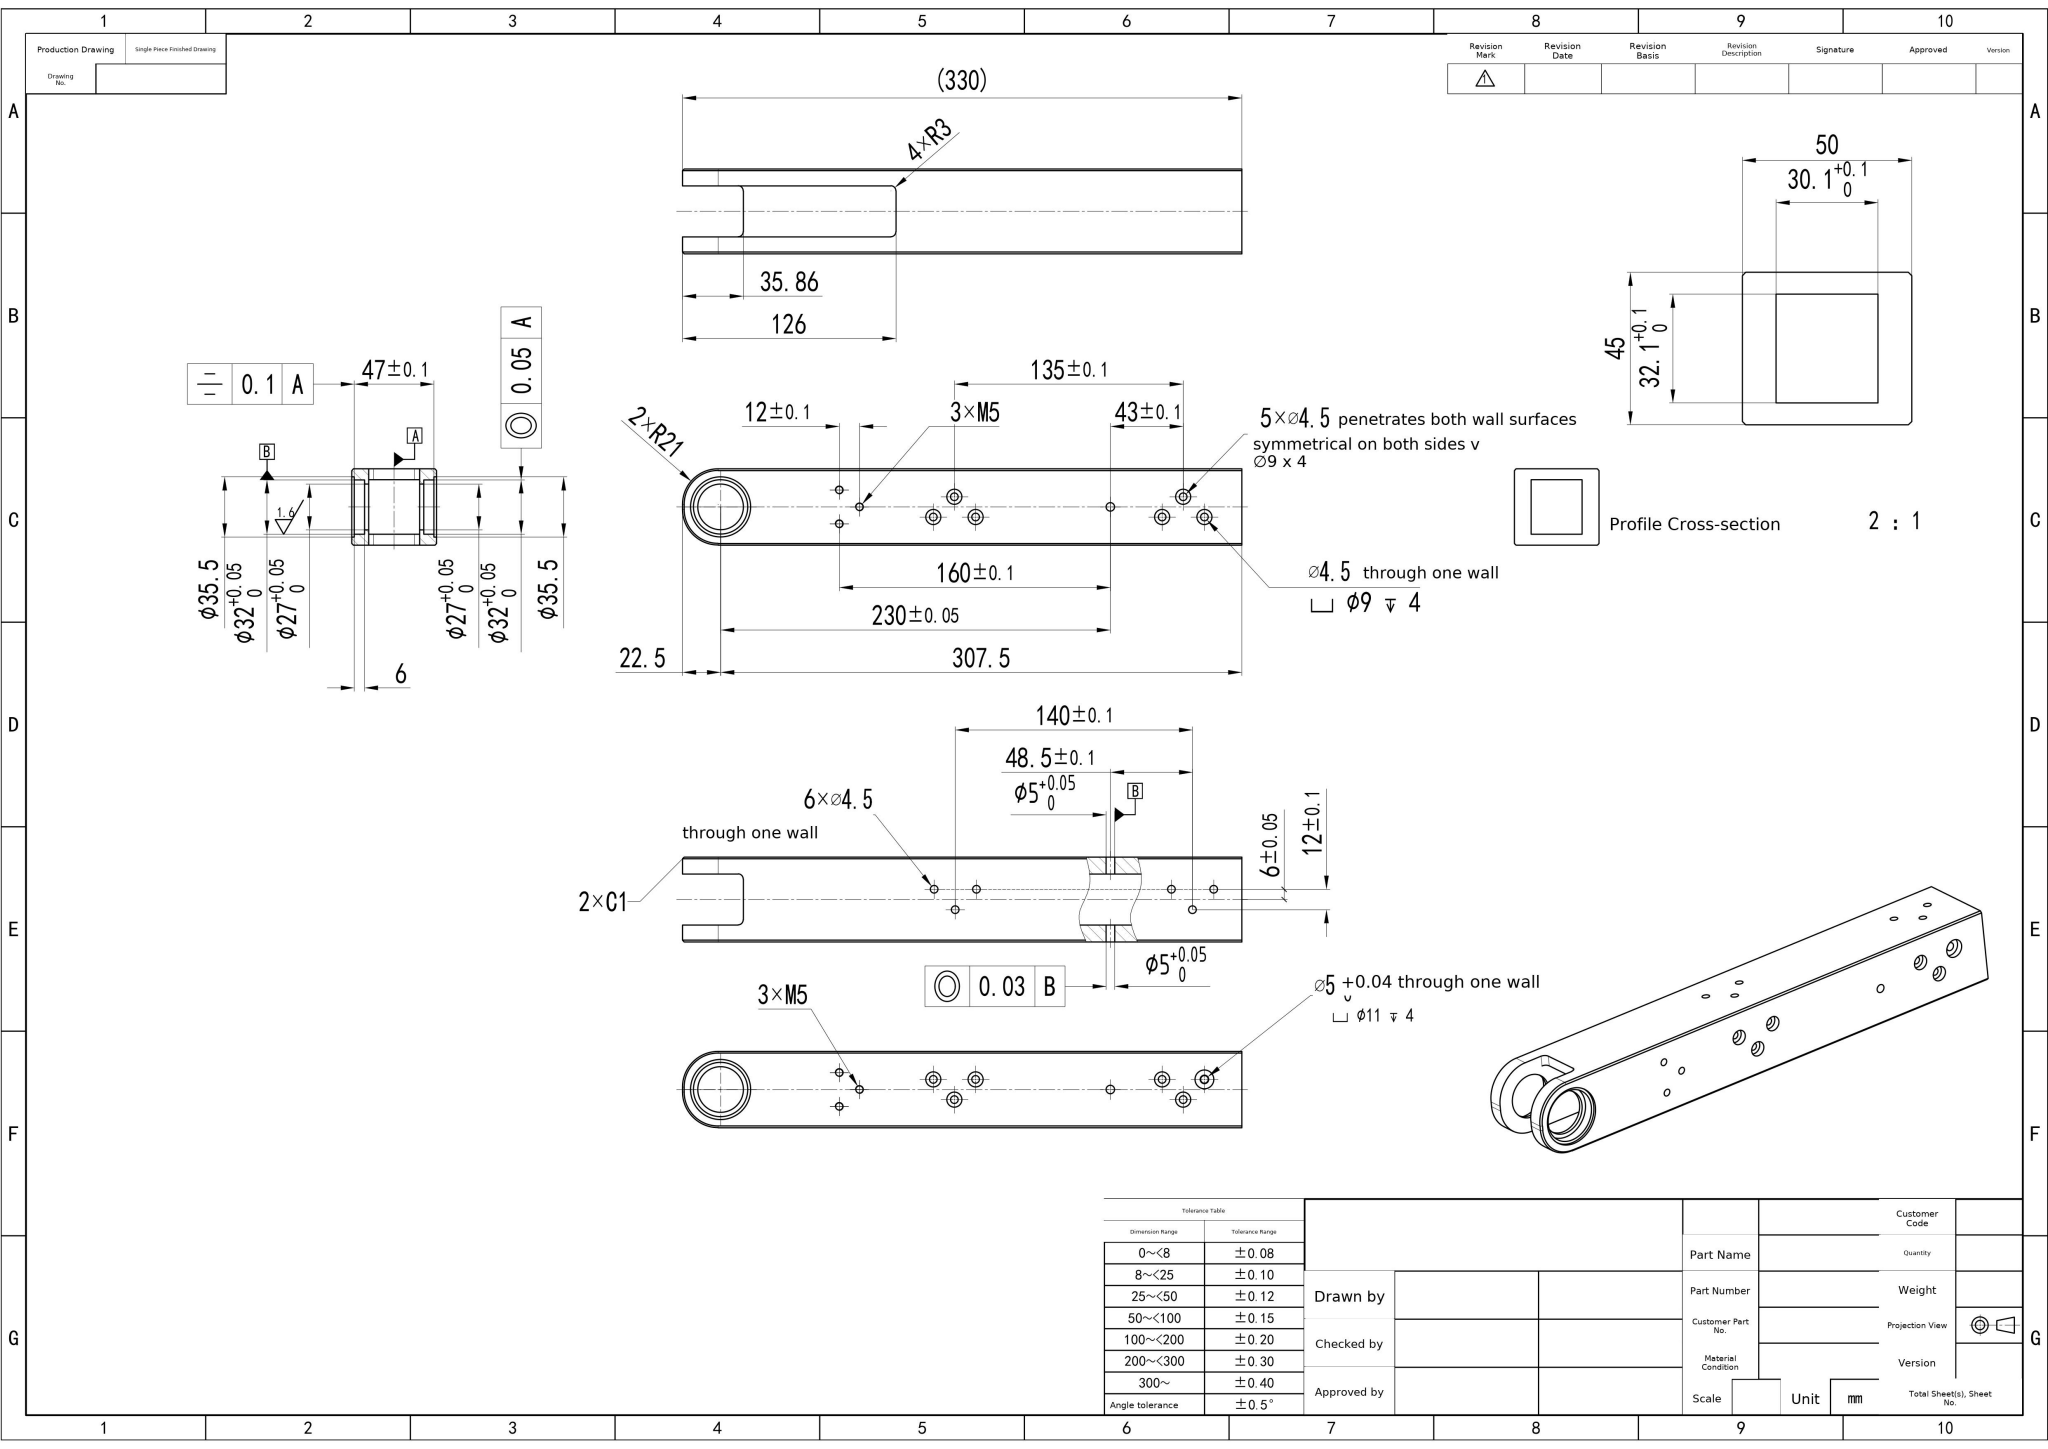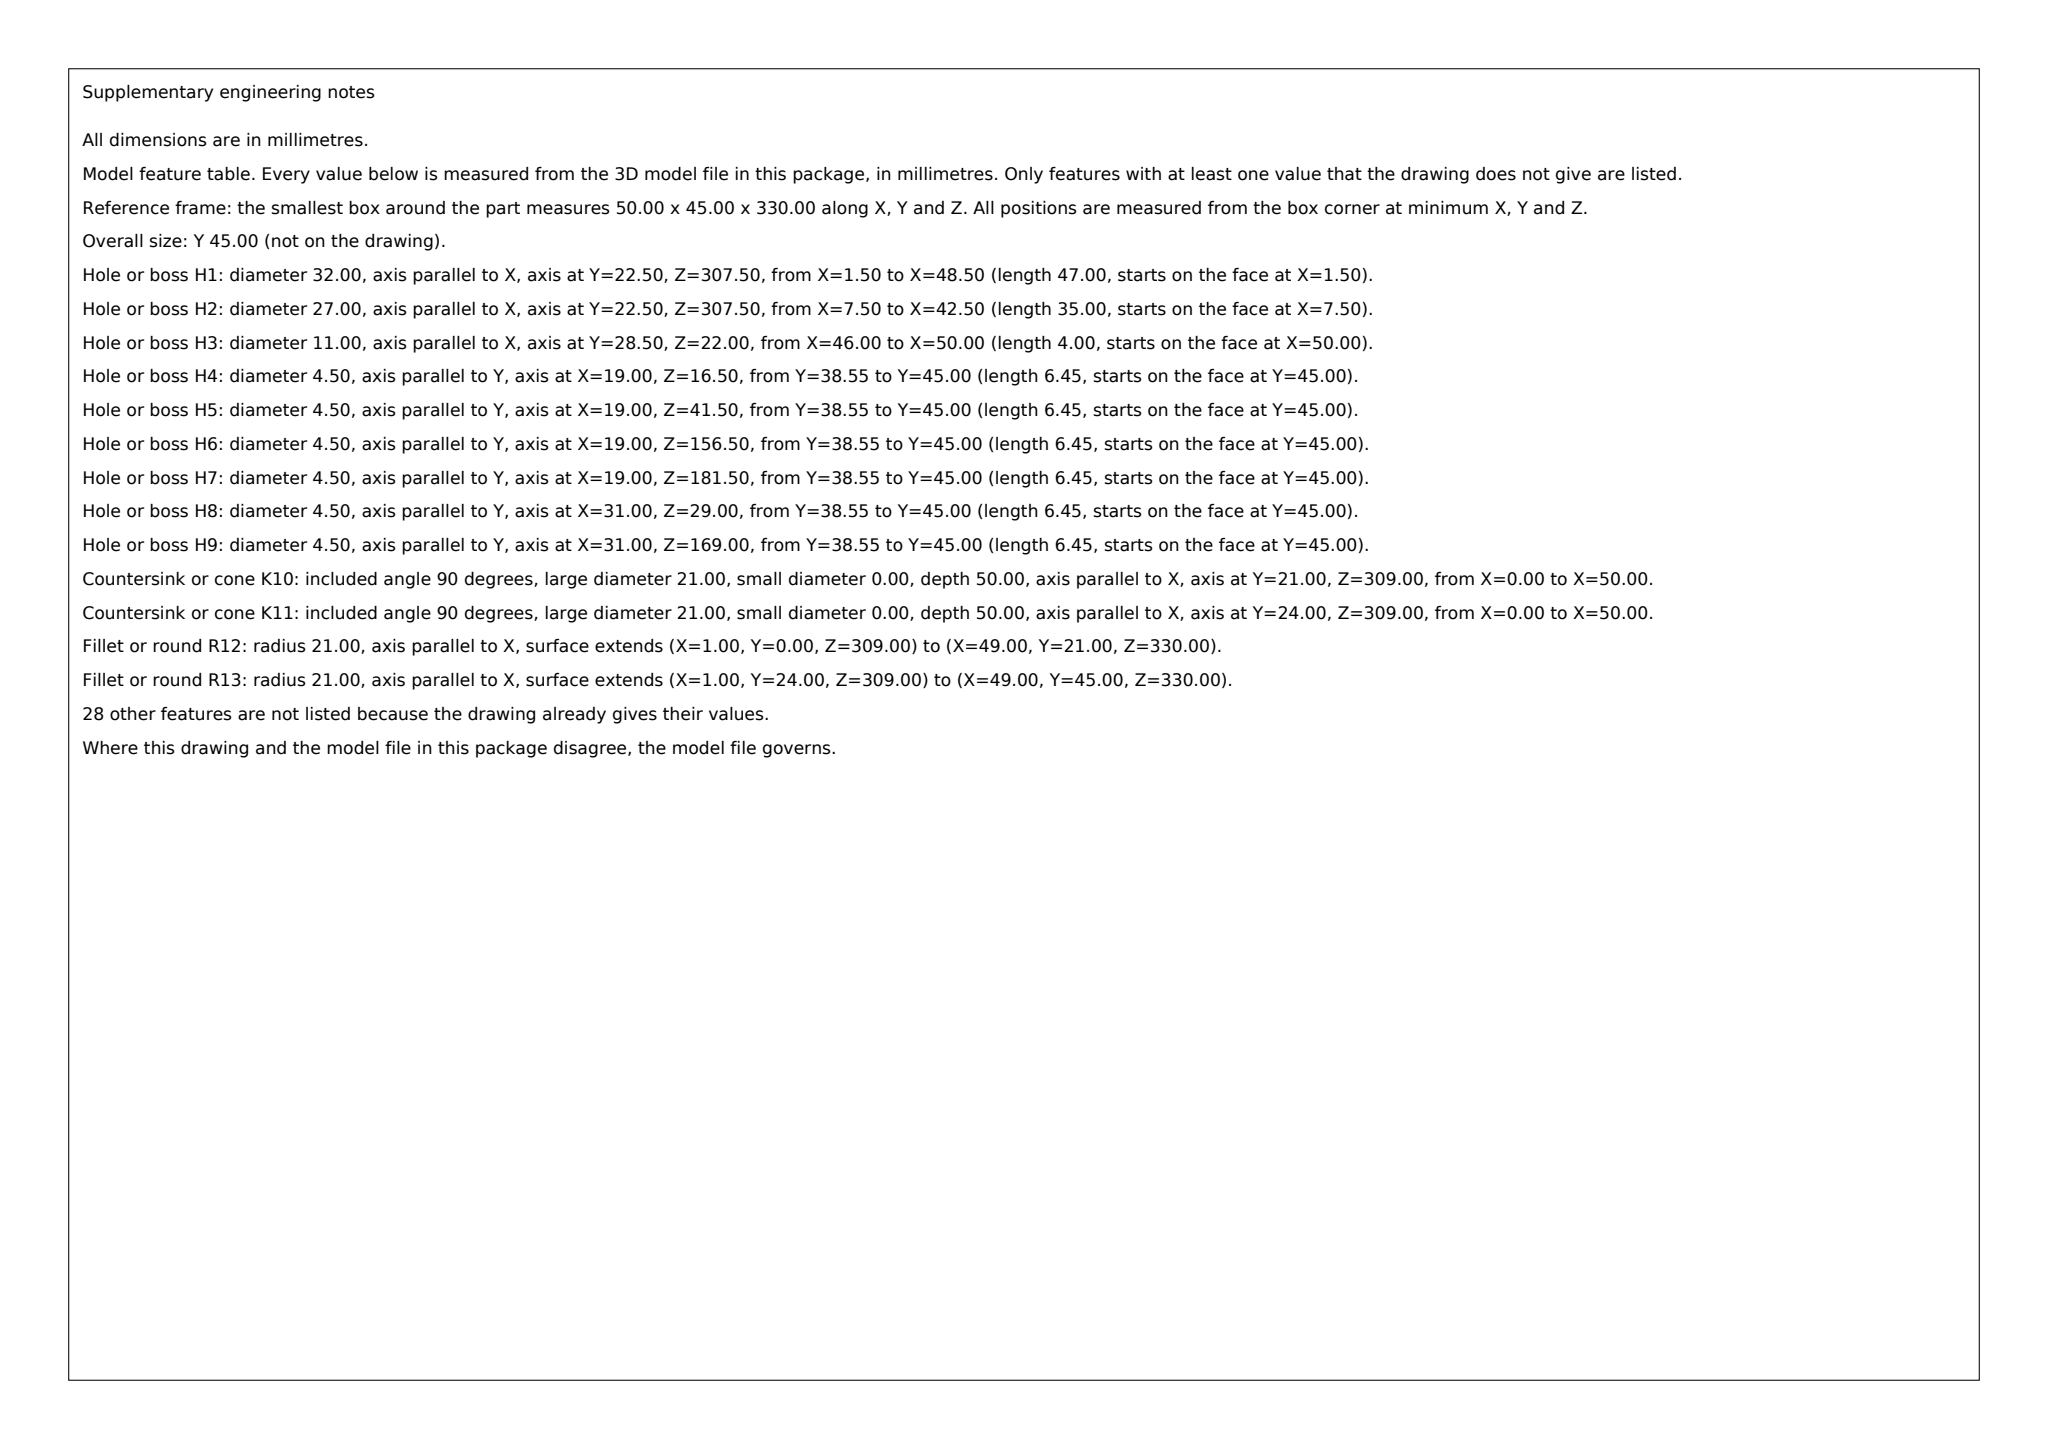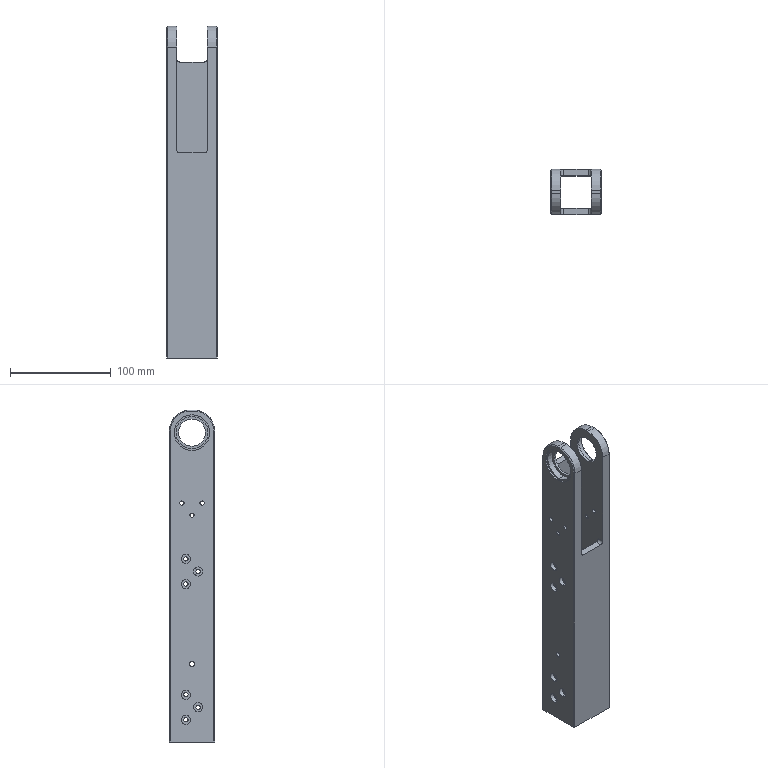Part | SolidWorks | mm | 1 solid | 135 faces | box 50 x 45 x 330 mm | volume 366362 mm3 | cylinder 96 | plane 35 | cone 4 | commonest cylinder face diameters 4.2 x34 9 x22 4.5 x12 5 x6 27 x4 35.5 x4 32 x4 6 x4